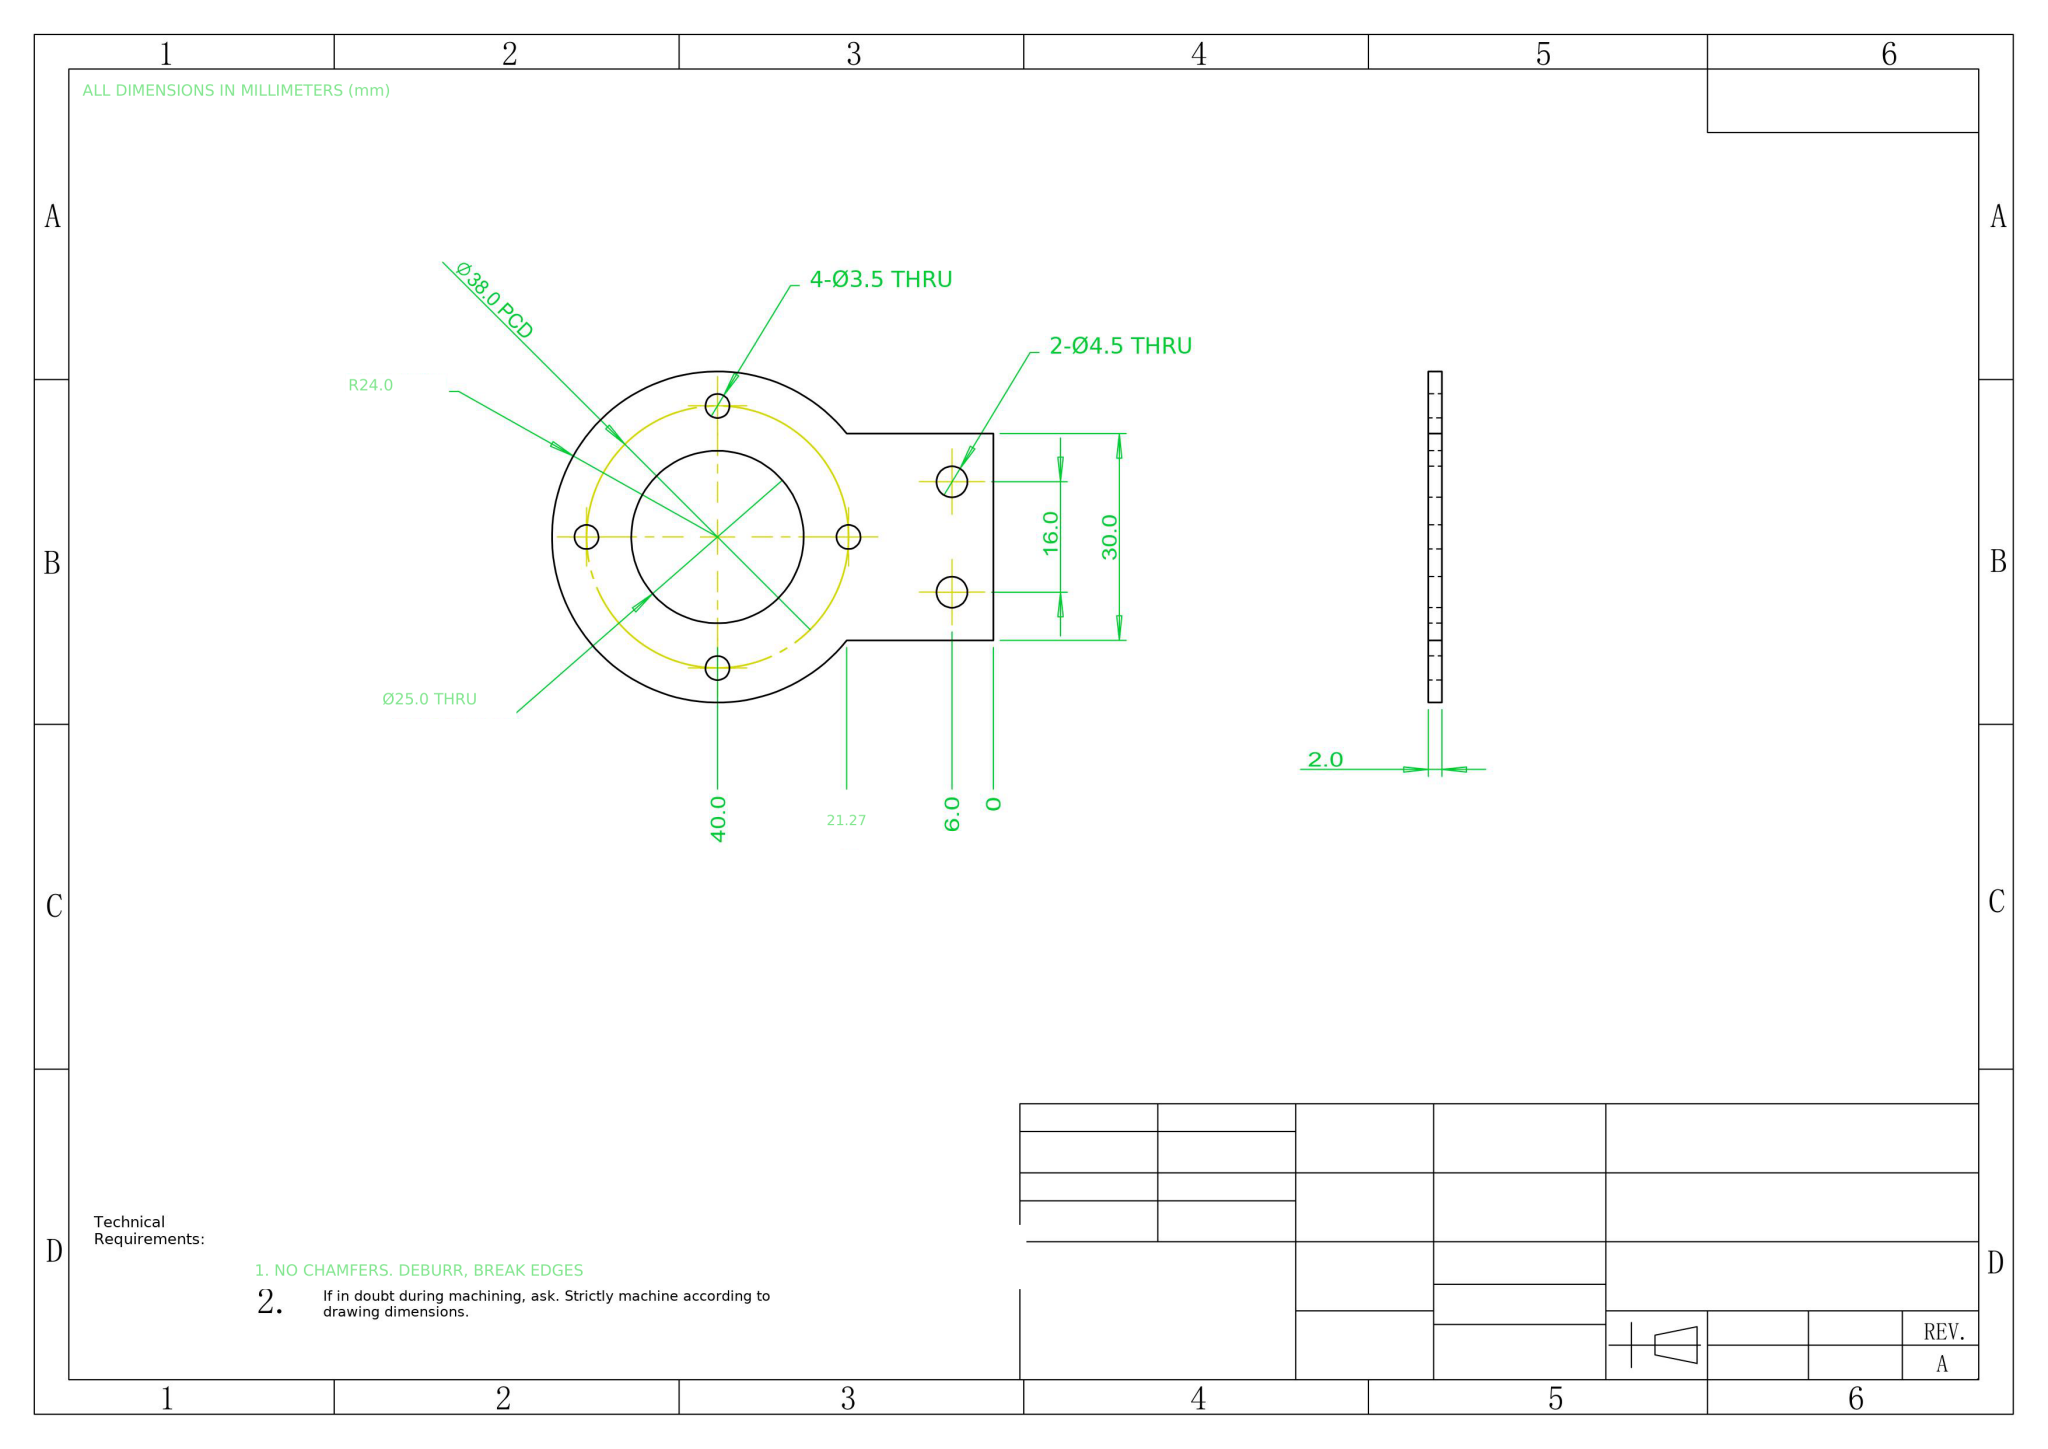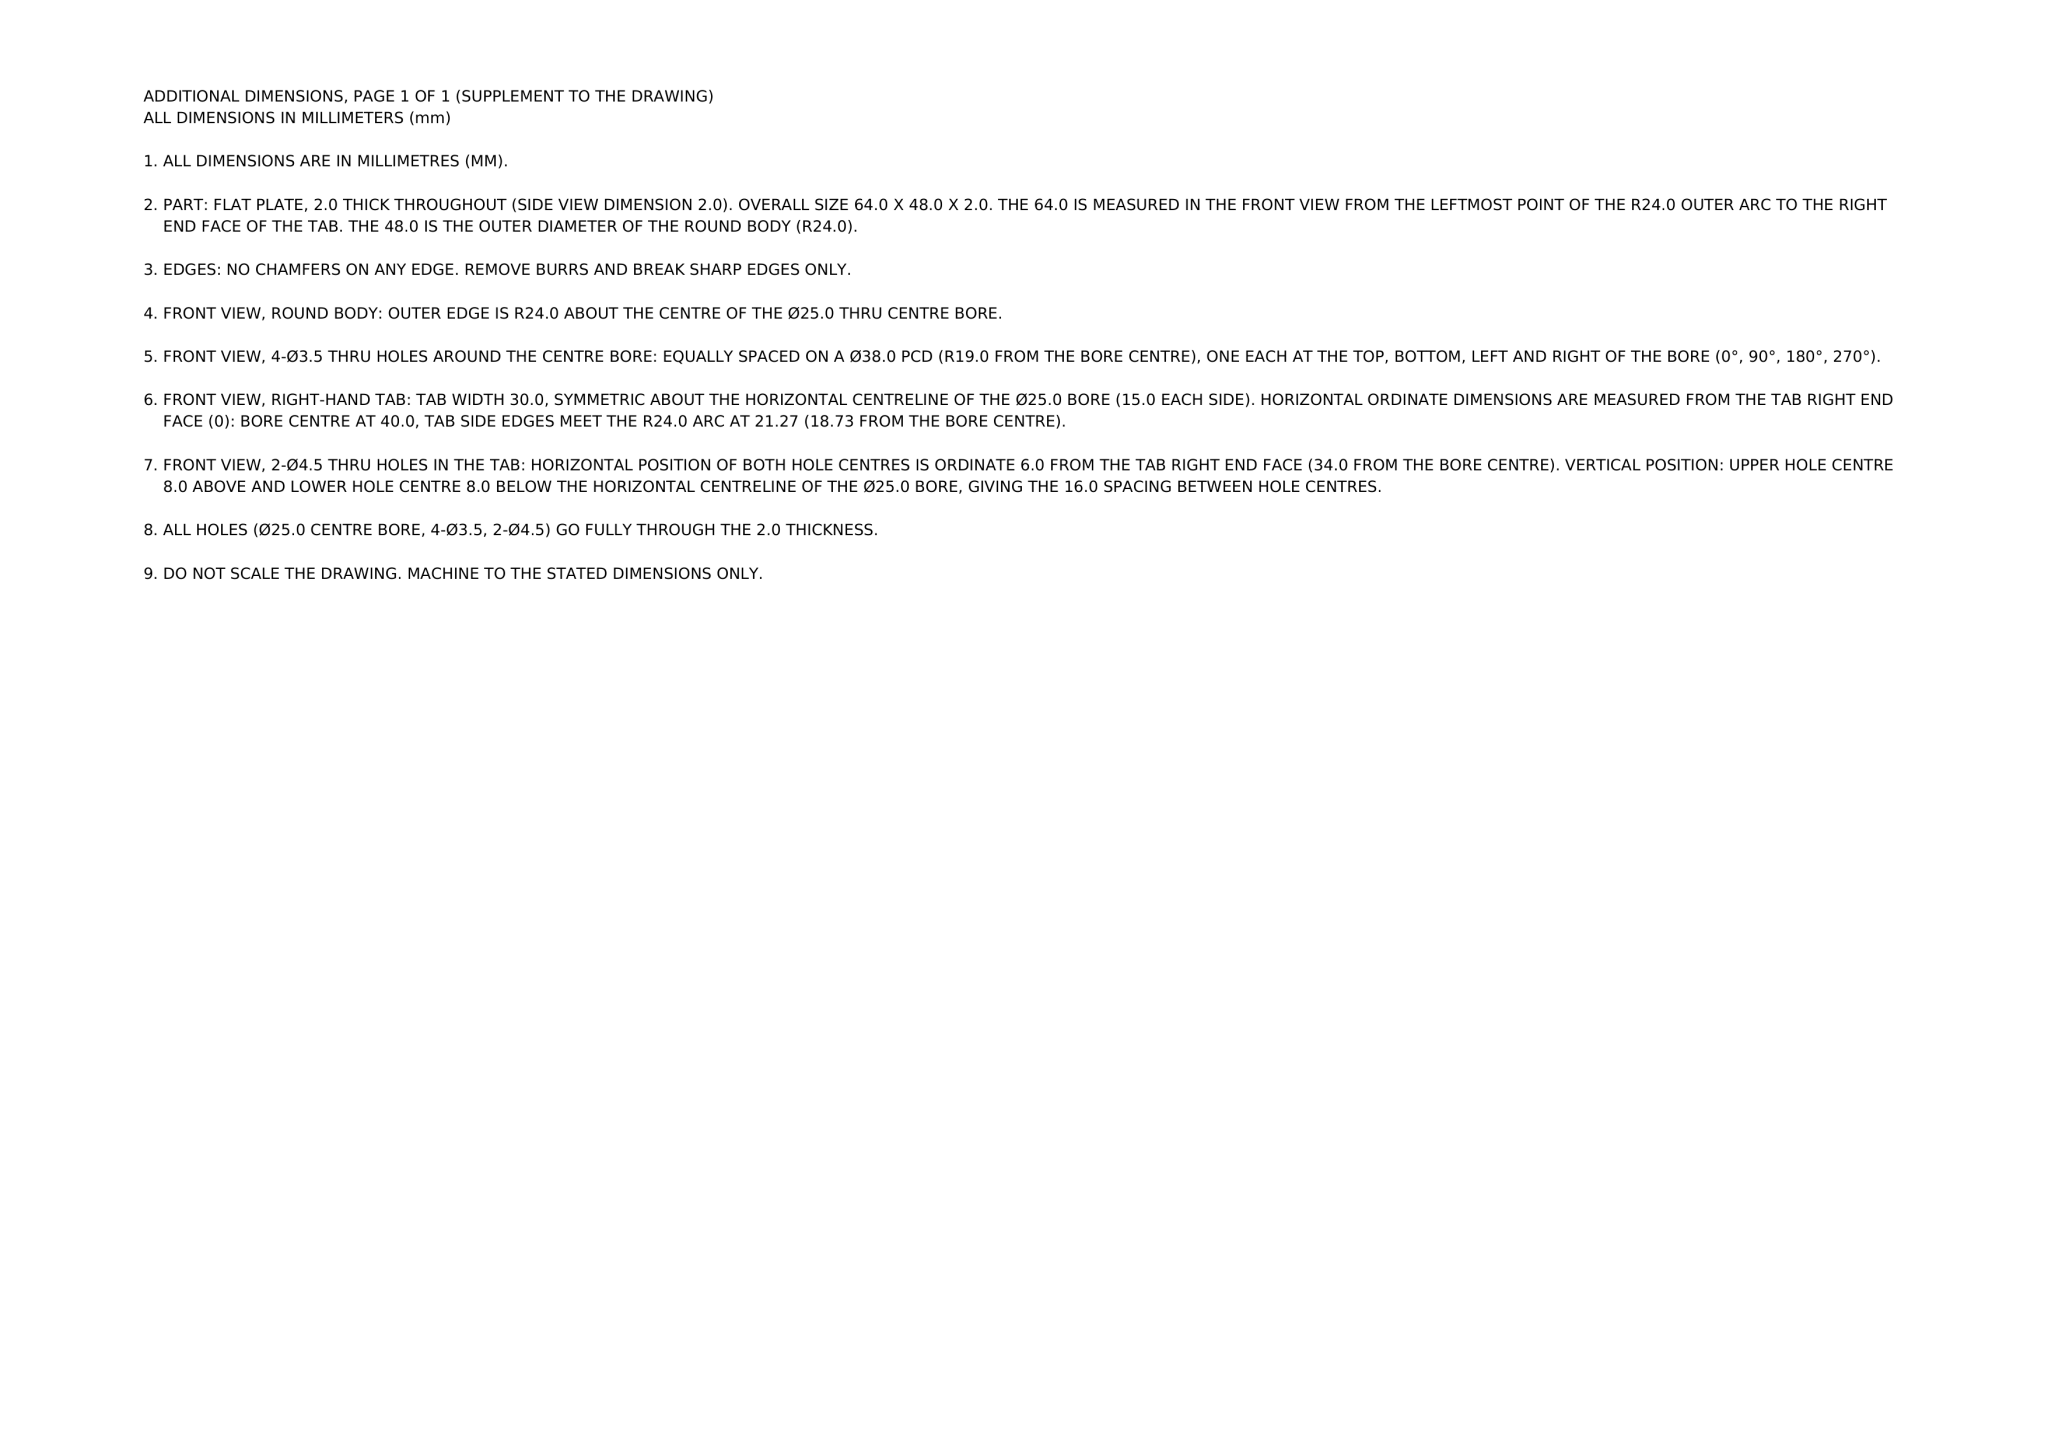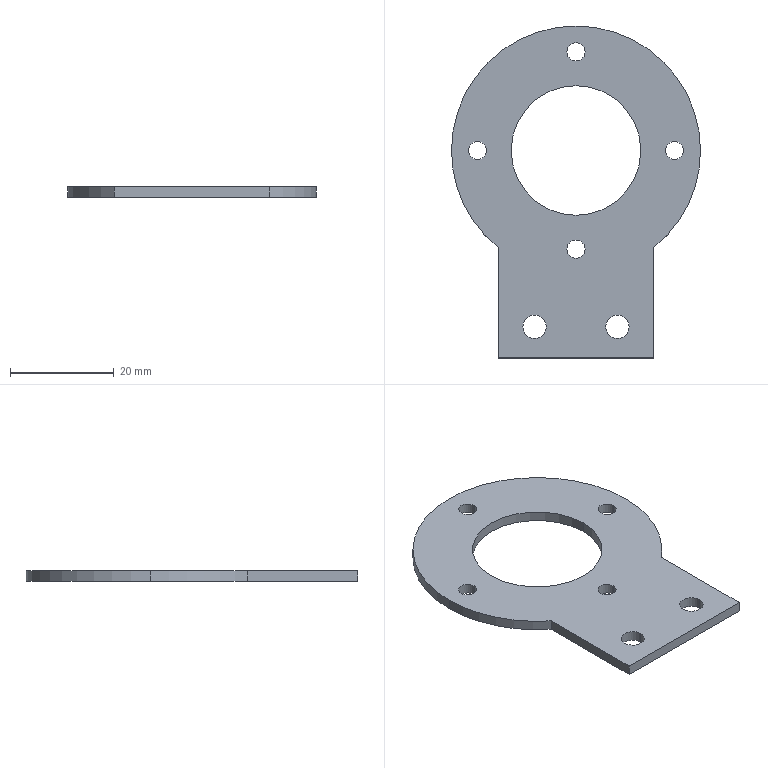Part | NX | mm | 1 solid | 22 faces | box 48 x 64 x 2 mm | volume 3557 mm3 | cylinder 17 | plane 5 | commonest cylinder face diameters 3.5 x8 4.5 x4 48 x3 25 x2
STEP:
#1=COLOUR_RGB('',0.5843,1.,0.);
#2=FILL_AREA_STYLE_COLOUR('',#1);
#3=FILL_AREA_STYLE('',(#2));
#4=SURFACE_STYLE_FILL_AREA(#3);
#5=SURFACE_SIDE_STYLE('',(#4));
#6=SURFACE_STYLE_USAGE(.BOTH.,#5);
#7=PRESENTATION_STYLE_ASSIGNMENT((#6));
#8=CARTESIAN_POINT('',(-10.25,-34.,0.));
#9=VERTEX_POINT('',#8);
#10=CARTESIAN_POINT('',(-5.75,-34.,0.));
#11=VERTEX_POINT('',#10);
#12=CARTESIAN_POINT('',(-8.,-34.,0.));
#13=DIRECTION('',(0.,0.,1.));
#14=DIRECTION('',(1.,0.,0.));
#15=AXIS2_PLACEMENT_3D('',#12,#13,#14);
#16=CIRCLE('',#15,2.25);
#17=EDGE_CURVE('',#9,#11,#16,.T.);
#18=ORIENTED_EDGE('',*,*,#17,.F.);
#19=CARTESIAN_POINT('',(-10.25,-34.,2.));
#20=VERTEX_POINT('',#19);
#21=CARTESIAN_POINT('',(-10.25,-34.,-8.));
#22=DIRECTION('',(0.,0.,1.));
#23=VECTOR('',#22,1000.);
#24=LINE('',#21,#23);
#25=EDGE_CURVE('',#9,#20,#24,.T.);
#26=ORIENTED_EDGE('',*,*,#25,.T.);
#27=CARTESIAN_POINT('',(-5.75,-34.,2.));
#28=VERTEX_POINT('',#27);
#29=CARTESIAN_POINT('',(-8.,-34.,2.));
#30=DIRECTION('',(0.,0.,1.));
#31=DIRECTION('',(-1.,0.,0.));
#32=AXIS2_PLACEMENT_3D('',#29,#30,#31);
#33=CIRCLE('',#32,2.25);
#34=EDGE_CURVE('',#20,#28,#33,.T.);
#35=ORIENTED_EDGE('',*,*,#34,.T.);
#36=CARTESIAN_POINT('',(-5.75,-34.,-8.));
#37=DIRECTION('',(0.,0.,1.));
#38=VECTOR('',#37,1000.);
#39=LINE('',#36,#38);
#40=EDGE_CURVE('',#11,#28,#39,.T.);
#41=ORIENTED_EDGE('',*,*,#40,.F.);
#42=EDGE_LOOP('',(#18,#26,#35,#41));
#43=FACE_OUTER_BOUND('',#42,.T.);
#44=CARTESIAN_POINT('',(-8.,-34.,-8.));
#45=DIRECTION('',(0.,0.,1.));
#46=DIRECTION('',(1.,0.,0.));
#47=AXIS2_PLACEMENT_3D('',#44,#45,#46);
#48=CYLINDRICAL_SURFACE('',#47,2.25);
#49=ADVANCED_FACE('',(#43),#48,.F.);
#50=CARTESIAN_POINT('',(5.75,-34.,0.));
#51=VERTEX_POINT('',#50);
#52=CARTESIAN_POINT('',(10.25,-34.,0.));
#53=VERTEX_POINT('',#52);
#54=CARTESIAN_POINT('',(8.,-34.,0.));
#55=DIRECTION('',(0.,0.,1.));
#56=DIRECTION('',(1.,0.,0.));
#57=AXIS2_PLACEMENT_3D('',#54,#55,#56);
#58=CIRCLE('',#57,2.25);
#59=EDGE_CURVE('',#51,#53,#58,.T.);
#60=ORIENTED_EDGE('',*,*,#59,.F.);
#61=CARTESIAN_POINT('',(5.75,-34.,2.));
#62=VERTEX_POINT('',#61);
#63=CARTESIAN_POINT('',(5.75,-34.,-8.));
#64=DIRECTION('',(0.,0.,1.));
#65=VECTOR('',#64,1000.);
#66=LINE('',#63,#65);
#67=EDGE_CURVE('',#51,#62,#66,.T.);
#68=ORIENTED_EDGE('',*,*,#67,.T.);
#69=CARTESIAN_POINT('',(10.25,-34.,2.));
#70=VERTEX_POINT('',#69);
#71=CARTESIAN_POINT('',(8.,-34.,2.));
#72=DIRECTION('',(0.,0.,1.));
#73=DIRECTION('',(1.,0.,0.));
#74=AXIS2_PLACEMENT_3D('',#71,#72,#73);
#75=CIRCLE('',#74,2.25);
#76=EDGE_CURVE('',#62,#70,#75,.T.);
#77=ORIENTED_EDGE('',*,*,#76,.T.);
#78=CARTESIAN_POINT('',(10.25,-34.,-8.));
#79=DIRECTION('',(0.,0.,1.));
#80=VECTOR('',#79,1000.);
#81=LINE('',#78,#80);
#82=EDGE_CURVE('',#53,#70,#81,.T.);
#83=ORIENTED_EDGE('',*,*,#82,.F.);
#84=EDGE_LOOP('',(#60,#68,#77,#83));
#85=FACE_OUTER_BOUND('',#84,.T.);
#86=CARTESIAN_POINT('',(8.,-34.,-8.));
#87=DIRECTION('',(0.,0.,1.));
#88=DIRECTION('',(1.,0.,0.));
#89=AXIS2_PLACEMENT_3D('',#86,#87,#88);
#90=CYLINDRICAL_SURFACE('',#89,2.25);
#91=ADVANCED_FACE('',(#85),#90,.F.);
#92=CARTESIAN_POINT('',(-20.75,0.,0.));
#93=VERTEX_POINT('',#92);
#94=CARTESIAN_POINT('',(-17.25,0.,0.));
#95=VERTEX_POINT('',#94);
#96=CARTESIAN_POINT('',(-19.,0.,0.));
#97=DIRECTION('',(0.,0.,1.));
#98=DIRECTION('',(1.,0.,0.));
#99=AXIS2_PLACEMENT_3D('',#96,#97,#98);
#100=CIRCLE('',#99,1.75);
#101=EDGE_CURVE('',#93,#95,#100,.T.);
#102=ORIENTED_EDGE('',*,*,#101,.F.);
#103=CARTESIAN_POINT('',(-20.75,0.,2.));
#104=VERTEX_POINT('',#103);
#105=CARTESIAN_POINT('',(-20.75,0.,0.));
#106=DIRECTION('',(0.,0.,1.));
#107=VECTOR('',#106,1000.);
#108=LINE('',#105,#107);
#109=EDGE_CURVE('',#93,#104,#108,.T.);
#110=ORIENTED_EDGE('',*,*,#109,.T.);
#111=CARTESIAN_POINT('',(-17.25,0.,2.));
#112=VERTEX_POINT('',#111);
#113=CARTESIAN_POINT('',(-19.,0.,2.));
#114=DIRECTION('',(0.,0.,1.));
#115=DIRECTION('',(1.,0.,0.));
#116=AXIS2_PLACEMENT_3D('',#113,#114,#115);
#117=CIRCLE('',#116,1.75);
#118=EDGE_CURVE('',#104,#112,#117,.T.);
#119=ORIENTED_EDGE('',*,*,#118,.T.);
#120=CARTESIAN_POINT('',(-17.25,0.,0.));
#121=DIRECTION('',(0.,0.,1.));
#122=VECTOR('',#121,1000.);
#123=LINE('',#120,#122);
#124=EDGE_CURVE('',#95,#112,#123,.T.);
#125=ORIENTED_EDGE('',*,*,#124,.F.);
#126=EDGE_LOOP('',(#102,#110,#119,#125));
#127=FACE_OUTER_BOUND('',#126,.T.);
#128=CARTESIAN_POINT('',(-19.,0.,0.));
#129=DIRECTION('',(0.,0.,1.));
#130=DIRECTION('',(1.,0.,0.));
#131=AXIS2_PLACEMENT_3D('',#128,#129,#130);
#132=CYLINDRICAL_SURFACE('',#131,1.75);
#133=ADVANCED_FACE('',(#127),#132,.F.);
#134=CARTESIAN_POINT('',(-1.75,-19.,0.));
#135=VERTEX_POINT('',#134);
#136=CARTESIAN_POINT('',(1.75,-19.,0.));
#137=VERTEX_POINT('',#136);
#138=CARTESIAN_POINT('',(0.,-19.,0.));
#139=DIRECTION('',(0.,0.,1.));
#140=DIRECTION('',(1.,0.,0.));
#141=AXIS2_PLACEMENT_3D('',#138,#139,#140);
#142=CIRCLE('',#141,1.75);
#143=EDGE_CURVE('',#135,#137,#142,.T.);
#144=ORIENTED_EDGE('',*,*,#143,.F.);
#145=CARTESIAN_POINT('',(-1.75,-19.,2.));
#146=VERTEX_POINT('',#145);
#147=CARTESIAN_POINT('',(-1.75,-19.,0.));
#148=DIRECTION('',(0.,0.,1.));
#149=VECTOR('',#148,1000.);
#150=LINE('',#147,#149);
#151=EDGE_CURVE('',#135,#146,#150,.T.);
#152=ORIENTED_EDGE('',*,*,#151,.T.);
#153=CARTESIAN_POINT('',(1.75,-19.,2.));
#154=VERTEX_POINT('',#153);
#155=CARTESIAN_POINT('',(0.,-19.,2.));
#156=DIRECTION('',(0.,0.,1.));
#157=DIRECTION('',(1.,0.,0.));
#158=AXIS2_PLACEMENT_3D('',#155,#156,#157);
#159=CIRCLE('',#158,1.75);
#160=EDGE_CURVE('',#146,#154,#159,.T.);
#161=ORIENTED_EDGE('',*,*,#160,.T.);
#162=CARTESIAN_POINT('',(1.75,-19.,0.));
#163=DIRECTION('',(0.,0.,1.));
#164=VECTOR('',#163,1000.);
#165=LINE('',#162,#164);
#166=EDGE_CURVE('',#137,#154,#165,.T.);
#167=ORIENTED_EDGE('',*,*,#166,.F.);
#168=EDGE_LOOP('',(#144,#152,#161,#167));
#169=FACE_OUTER_BOUND('',#168,.T.);
#170=CARTESIAN_POINT('',(0.,-19.,0.));
#171=DIRECTION('',(0.,0.,1.));
#172=DIRECTION('',(1.,0.,0.));
#173=AXIS2_PLACEMENT_3D('',#170,#171,#172);
#174=CYLINDRICAL_SURFACE('',#173,1.75);
#175=ADVANCED_FACE('',(#169),#174,.F.);
#176=CARTESIAN_POINT('',(17.25,0.,0.));
#177=VERTEX_POINT('',#176);
#178=CARTESIAN_POINT('',(20.75,0.,0.));
#179=VERTEX_POINT('',#178);
#180=CARTESIAN_POINT('',(19.,0.,0.));
#181=DIRECTION('',(0.,0.,1.));
#182=DIRECTION('',(1.,0.,0.));
#183=AXIS2_PLACEMENT_3D('',#180,#181,#182);
#184=CIRCLE('',#183,1.75);
#185=EDGE_CURVE('',#177,#179,#184,.T.);
#186=ORIENTED_EDGE('',*,*,#185,.F.);
#187=CARTESIAN_POINT('',(17.25,0.,2.));
#188=VERTEX_POINT('',#187);
#189=CARTESIAN_POINT('',(17.25,0.,0.));
#190=DIRECTION('',(0.,0.,1.));
#191=VECTOR('',#190,1000.);
#192=LINE('',#189,#191);
#193=EDGE_CURVE('',#177,#188,#192,.T.);
#194=ORIENTED_EDGE('',*,*,#193,.T.);
#195=CARTESIAN_POINT('',(20.75,0.,2.));
#196=VERTEX_POINT('',#195);
#197=CARTESIAN_POINT('',(19.,0.,2.));
#198=DIRECTION('',(0.,0.,1.));
#199=DIRECTION('',(1.,0.,0.));
#200=AXIS2_PLACEMENT_3D('',#197,#198,#199);
#201=CIRCLE('',#200,1.75);
#202=EDGE_CURVE('',#188,#196,#201,.T.);
#203=ORIENTED_EDGE('',*,*,#202,.T.);
#204=CARTESIAN_POINT('',(20.75,0.,0.));
#205=DIRECTION('',(0.,0.,1.));
#206=VECTOR('',#205,1000.);
#207=LINE('',#204,#206);
#208=EDGE_CURVE('',#179,#196,#207,.T.);
#209=ORIENTED_EDGE('',*,*,#208,.F.);
#210=EDGE_LOOP('',(#186,#194,#203,#209));
#211=FACE_OUTER_BOUND('',#210,.T.);
#212=CARTESIAN_POINT('',(19.,0.,0.));
#213=DIRECTION('',(0.,0.,1.));
#214=DIRECTION('',(1.,0.,0.));
#215=AXIS2_PLACEMENT_3D('',#212,#213,#214);
#216=CYLINDRICAL_SURFACE('',#215,1.75);
#217=ADVANCED_FACE('',(#211),#216,.F.);
#218=CARTESIAN_POINT('',(-1.75,19.,0.));
#219=VERTEX_POINT('',#218);
#220=CARTESIAN_POINT('',(1.75,19.,0.));
#221=VERTEX_POINT('',#220);
#222=CARTESIAN_POINT('',(0.,19.,0.));
#223=DIRECTION('',(0.,0.,1.));
#224=DIRECTION('',(1.,0.,0.));
#225=AXIS2_PLACEMENT_3D('',#222,#223,#224);
#226=CIRCLE('',#225,1.75);
#227=EDGE_CURVE('',#219,#221,#226,.T.);
#228=ORIENTED_EDGE('',*,*,#227,.F.);
#229=CARTESIAN_POINT('',(-1.75,19.,2.));
#230=VERTEX_POINT('',#229);
#231=CARTESIAN_POINT('',(-1.75,19.,0.));
#232=DIRECTION('',(0.,0.,1.));
#233=VECTOR('',#232,1000.);
#234=LINE('',#231,#233);
#235=EDGE_CURVE('',#219,#230,#234,.T.);
#236=ORIENTED_EDGE('',*,*,#235,.T.);
#237=CARTESIAN_POINT('',(1.75,19.,2.));
#238=VERTEX_POINT('',#237);
#239=CARTESIAN_POINT('',(0.,19.,2.));
#240=DIRECTION('',(0.,0.,1.));
#241=DIRECTION('',(1.,0.,0.));
#242=AXIS2_PLACEMENT_3D('',#239,#240,#241);
#243=CIRCLE('',#242,1.75);
#244=EDGE_CURVE('',#230,#238,#243,.T.);
#245=ORIENTED_EDGE('',*,*,#244,.T.);
#246=CARTESIAN_POINT('',(1.75,19.,0.));
#247=DIRECTION('',(0.,0.,1.));
#248=VECTOR('',#247,1000.);
#249=LINE('',#246,#248);
#250=EDGE_CURVE('',#221,#238,#249,.T.);
#251=ORIENTED_EDGE('',*,*,#250,.F.);
#252=EDGE_LOOP('',(#228,#236,#245,#251));
#253=FACE_OUTER_BOUND('',#252,.T.);
#254=CARTESIAN_POINT('',(0.,19.,0.));
#255=DIRECTION('',(0.,0.,1.));
#256=DIRECTION('',(1.,0.,0.));
#257=AXIS2_PLACEMENT_3D('',#254,#255,#256);
#258=CYLINDRICAL_SURFACE('',#257,1.75);
#259=ADVANCED_FACE('',(#253),#258,.F.);
#260=CARTESIAN_POINT('',(-12.5,0.,2.));
#261=VERTEX_POINT('',#260);
#262=CARTESIAN_POINT('',(12.5,0.,2.));
#263=VERTEX_POINT('',#262);
#264=CARTESIAN_POINT('',(0.,0.,2.));
#265=DIRECTION('',(0.,0.,1.));
#266=DIRECTION('',(1.,0.,0.));
#267=AXIS2_PLACEMENT_3D('',#264,#265,#266);
#268=CIRCLE('',#267,12.5);
#269=EDGE_CURVE('',#261,#263,#268,.T.);
#270=ORIENTED_EDGE('',*,*,#269,.T.);
#271=CARTESIAN_POINT('',(12.5,0.,0.));
#272=VERTEX_POINT('',#271);
#273=CARTESIAN_POINT('',(12.5,0.,2.));
#274=DIRECTION('',(0.,0.,-1.));
#275=VECTOR('',#274,1000.);
#276=LINE('',#273,#275);
#277=EDGE_CURVE('',#263,#272,#276,.T.);
#278=ORIENTED_EDGE('',*,*,#277,.T.);
#279=CARTESIAN_POINT('',(-12.5,0.,0.));
#280=VERTEX_POINT('',#279);
#281=CARTESIAN_POINT('',(0.,0.,0.));
#282=DIRECTION('',(0.,0.,1.));
#283=DIRECTION('',(1.,0.,0.));
#284=AXIS2_PLACEMENT_3D('',#281,#282,#283);
#285=CIRCLE('',#284,12.5);
#286=EDGE_CURVE('',#280,#272,#285,.T.);
#287=ORIENTED_EDGE('',*,*,#286,.F.);
#288=CARTESIAN_POINT('',(-12.5,0.,2.));
#289=DIRECTION('',(0.,0.,-1.));
#290=VECTOR('',#289,1000.);
#291=LINE('',#288,#290);
#292=EDGE_CURVE('',#261,#280,#291,.T.);
#293=ORIENTED_EDGE('',*,*,#292,.F.);
#294=EDGE_LOOP('',(#270,#278,#287,#293));
#295=FACE_OUTER_BOUND('',#294,.T.);
#296=CARTESIAN_POINT('',(0.,0.,2.));
#297=DIRECTION('',(0.,0.,-1.));
#298=DIRECTION('',(-1.,0.,0.));
#299=AXIS2_PLACEMENT_3D('',#296,#297,#298);
#300=CYLINDRICAL_SURFACE('',#299,12.5);
#301=ADVANCED_FACE('',(#295),#300,.F.);
#302=CARTESIAN_POINT('',(24.,0.,2.));
#303=VERTEX_POINT('',#302);
#304=CARTESIAN_POINT('',(-24.,0.,2.));
#305=VERTEX_POINT('',#304);
#306=CARTESIAN_POINT('',(0.,0.,2.));
#307=DIRECTION('',(0.,0.,1.));
#308=DIRECTION('',(1.,0.,0.));
#309=AXIS2_PLACEMENT_3D('',#306,#307,#308);
#310=CIRCLE('',#309,24.);
#311=EDGE_CURVE('',#303,#305,#310,.T.);
#312=ORIENTED_EDGE('',*,*,#311,.F.);
#313=CARTESIAN_POINT('',(24.,0.,0.));
#314=VERTEX_POINT('',#313);
#315=CARTESIAN_POINT('',(24.,0.,2.));
#316=DIRECTION('',(0.,0.,-1.));
#317=VECTOR('',#316,1000.);
#318=LINE('',#315,#317);
#319=EDGE_CURVE('',#303,#314,#318,.T.);
#320=ORIENTED_EDGE('',*,*,#319,.T.);
#321=CARTESIAN_POINT('',(-24.,0.,0.));
#322=VERTEX_POINT('',#321);
#323=CARTESIAN_POINT('',(0.,0.,0.));
#324=DIRECTION('',(0.,0.,1.));
#325=DIRECTION('',(1.,0.,0.));
#326=AXIS2_PLACEMENT_3D('',#323,#324,#325);
#327=CIRCLE('',#326,24.);
#328=EDGE_CURVE('',#314,#322,#327,.T.);
#329=ORIENTED_EDGE('',*,*,#328,.T.);
#330=CARTESIAN_POINT('',(-24.,0.,2.));
#331=DIRECTION('',(0.,0.,-1.));
#332=VECTOR('',#331,1000.);
#333=LINE('',#330,#332);
#334=EDGE_CURVE('',#305,#322,#333,.T.);
#335=ORIENTED_EDGE('',*,*,#334,.F.);
#336=EDGE_LOOP('',(#312,#320,#329,#335));
#337=FACE_OUTER_BOUND('',#336,.T.);
#338=CARTESIAN_POINT('',(0.,0.,2.));
#339=DIRECTION('',(0.,0.,-1.));
#340=DIRECTION('',(-1.,0.,0.));
#341=AXIS2_PLACEMENT_3D('',#338,#339,#340);
#342=CYLINDRICAL_SURFACE('',#341,24.);
#343=ADVANCED_FACE('',(#337),#342,.T.);
#344=CARTESIAN_POINT('',(-15.,-18.735,2.));
#345=VERTEX_POINT('',#344);
#346=CARTESIAN_POINT('',(0.,0.,2.));
#347=DIRECTION('',(0.,0.,1.));
#348=DIRECTION('',(1.,0.,0.));
#349=AXIS2_PLACEMENT_3D('',#346,#347,#348);
#350=CIRCLE('',#349,24.);
#351=EDGE_CURVE('',#305,#345,#350,.T.);
#352=ORIENTED_EDGE('',*,*,#351,.F.);
#353=ORIENTED_EDGE('',*,*,#334,.T.);
#354=CARTESIAN_POINT('',(-15.,-18.735,0.));
#355=VERTEX_POINT('',#354);
#356=CARTESIAN_POINT('',(0.,0.,0.));
#357=DIRECTION('',(0.,0.,1.));
#358=DIRECTION('',(1.,0.,0.));
#359=AXIS2_PLACEMENT_3D('',#356,#357,#358);
#360=CIRCLE('',#359,24.);
#361=EDGE_CURVE('',#322,#355,#360,.T.);
#362=ORIENTED_EDGE('',*,*,#361,.T.);
#363=CARTESIAN_POINT('',(-15.,-18.735,2.));
#364=DIRECTION('',(0.,0.,1.));
#365=VECTOR('',#364,1000.);
#366=LINE('',#363,#365);
#367=EDGE_CURVE('',#355,#345,#366,.T.);
#368=ORIENTED_EDGE('',*,*,#367,.T.);
#369=EDGE_LOOP('',(#352,#353,#362,#368));
#370=FACE_OUTER_BOUND('',#369,.T.);
#371=CARTESIAN_POINT('',(0.,0.,2.));
#372=DIRECTION('',(0.,0.,-1.));
#373=DIRECTION('',(-1.,0.,0.));
#374=AXIS2_PLACEMENT_3D('',#371,#372,#373);
#375=CYLINDRICAL_SURFACE('',#374,24.);
#376=ADVANCED_FACE('',(#370),#375,.T.);
#377=CARTESIAN_POINT('',(-8.,-34.,2.));
#378=DIRECTION('',(0.,0.,1.));
#379=DIRECTION('',(-1.,0.,0.));
#380=AXIS2_PLACEMENT_3D('',#377,#378,#379);
#381=CIRCLE('',#380,2.25);
#382=EDGE_CURVE('',#28,#20,#381,.T.);
#383=ORIENTED_EDGE('',*,*,#382,.F.);
#384=ORIENTED_EDGE('',*,*,#34,.F.);
#385=EDGE_LOOP('',(#383,#384));
#386=FACE_BOUND('',#385,.T.);
#387=CARTESIAN_POINT('',(8.,-34.,2.));
#388=DIRECTION('',(0.,0.,1.));
#389=DIRECTION('',(1.,0.,0.));
#390=AXIS2_PLACEMENT_3D('',#387,#388,#389);
#391=CIRCLE('',#390,2.25);
#392=EDGE_CURVE('',#70,#62,#391,.T.);
#393=ORIENTED_EDGE('',*,*,#392,.F.);
#394=ORIENTED_EDGE('',*,*,#76,.F.);
#395=EDGE_LOOP('',(#393,#394));
#396=FACE_BOUND('',#395,.T.);
#397=CARTESIAN_POINT('',(-19.,0.,2.));
#398=DIRECTION('',(0.,0.,1.));
#399=DIRECTION('',(1.,0.,0.));
#400=AXIS2_PLACEMENT_3D('',#397,#398,#399);
#401=CIRCLE('',#400,1.75);
#402=EDGE_CURVE('',#112,#104,#401,.T.);
#403=ORIENTED_EDGE('',*,*,#402,.F.);
#404=ORIENTED_EDGE('',*,*,#118,.F.);
#405=EDGE_LOOP('',(#403,#404));
#406=FACE_BOUND('',#405,.T.);
#407=CARTESIAN_POINT('',(0.,-19.,2.));
#408=DIRECTION('',(0.,0.,1.));
#409=DIRECTION('',(1.,0.,0.));
#410=AXIS2_PLACEMENT_3D('',#407,#408,#409);
#411=CIRCLE('',#410,1.75);
#412=EDGE_CURVE('',#154,#146,#411,.T.);
#413=ORIENTED_EDGE('',*,*,#412,.F.);
#414=ORIENTED_EDGE('',*,*,#160,.F.);
#415=EDGE_LOOP('',(#413,#414));
#416=FACE_BOUND('',#415,.T.);
#417=CARTESIAN_POINT('',(19.,0.,2.));
#418=DIRECTION('',(0.,0.,1.));
#419=DIRECTION('',(1.,0.,0.));
#420=AXIS2_PLACEMENT_3D('',#417,#418,#419);
#421=CIRCLE('',#420,1.75);
#422=EDGE_CURVE('',#196,#188,#421,.T.);
#423=ORIENTED_EDGE('',*,*,#422,.F.);
#424=ORIENTED_EDGE('',*,*,#202,.F.);
#425=EDGE_LOOP('',(#423,#424));
#426=FACE_BOUND('',#425,.T.);
#427=CARTESIAN_POINT('',(0.,19.,2.));
#428=DIRECTION('',(0.,0.,1.));
#429=DIRECTION('',(1.,0.,0.));
#430=AXIS2_PLACEMENT_3D('',#427,#428,#429);
#431=CIRCLE('',#430,1.75);
#432=EDGE_CURVE('',#238,#230,#431,.T.);
#433=ORIENTED_EDGE('',*,*,#432,.F.);
#434=ORIENTED_EDGE('',*,*,#244,.F.);
#435=EDGE_LOOP('',(#433,#434));
#436=FACE_BOUND('',#435,.T.);
#437=CARTESIAN_POINT('',(15.,-18.735,2.));
#438=VERTEX_POINT('',#437);
#439=CARTESIAN_POINT('',(0.,0.,2.));
#440=DIRECTION('',(0.,0.,1.));
#441=DIRECTION('',(1.,0.,0.));
#442=AXIS2_PLACEMENT_3D('',#439,#440,#441);
#443=CIRCLE('',#442,24.);
#444=EDGE_CURVE('',#438,#303,#443,.T.);
#445=ORIENTED_EDGE('',*,*,#444,.T.);
#446=ORIENTED_EDGE('',*,*,#311,.T.);
#447=ORIENTED_EDGE('',*,*,#351,.T.);
#448=CARTESIAN_POINT('',(-15.,-40.,2.));
#449=VERTEX_POINT('',#448);
#450=CARTESIAN_POINT('',(-15.,-15.209,2.));
#451=DIRECTION('',(0.,-1.,0.));
#452=VECTOR('',#451,1000.);
#453=LINE('',#450,#452);
#454=EDGE_CURVE('',#345,#449,#453,.T.);
#455=ORIENTED_EDGE('',*,*,#454,.T.);
#456=CARTESIAN_POINT('',(15.,-40.,2.));
#457=VERTEX_POINT('',#456);
#458=CARTESIAN_POINT('',(-15.,-40.,2.));
#459=DIRECTION('',(1.,0.,0.));
#460=VECTOR('',#459,1000.);
#461=LINE('',#458,#460);
#462=EDGE_CURVE('',#449,#457,#461,.T.);
#463=ORIENTED_EDGE('',*,*,#462,.T.);
#464=CARTESIAN_POINT('',(15.,-15.209,2.));
#465=DIRECTION('',(-0.,1.,0.));
#466=VECTOR('',#465,1000.);
#467=LINE('',#464,#466);
#468=EDGE_CURVE('',#457,#438,#467,.T.);
#469=ORIENTED_EDGE('',*,*,#468,.T.);
#470=EDGE_LOOP('',(#445,#446,#447,#455,#463,#469));
#471=FACE_OUTER_BOUND('',#470,.T.);
#472=ORIENTED_EDGE('',*,*,#269,.F.);
#473=CARTESIAN_POINT('',(0.,0.,2.));
#474=DIRECTION('',(0.,0.,1.));
#475=DIRECTION('',(1.,0.,0.));
#476=AXIS2_PLACEMENT_3D('',#473,#474,#475);
#477=CIRCLE('',#476,12.5);
#478=EDGE_CURVE('',#263,#261,#477,.T.);
#479=ORIENTED_EDGE('',*,*,#478,.F.);
#480=EDGE_LOOP('',(#472,#479));
#481=FACE_BOUND('',#480,.T.);
#482=CARTESIAN_POINT('',(0.,0.,2.));
#483=DIRECTION('',(0.,0.,1.));
#484=DIRECTION('',(1.,0.,0.));
#485=AXIS2_PLACEMENT_3D('',#482,#483,#484);
#486=PLANE('',#485);
#487=ADVANCED_FACE('',(#386,#396,#406,#416,#426,#436,#471,#481),#486,.T.);
#488=CARTESIAN_POINT('',(-8.,-34.,0.));
#489=DIRECTION('',(0.,0.,1.));
#490=DIRECTION('',(1.,0.,0.));
#491=AXIS2_PLACEMENT_3D('',#488,#489,#490);
#492=CIRCLE('',#491,2.25);
#493=EDGE_CURVE('',#11,#9,#492,.T.);
#494=ORIENTED_EDGE('',*,*,#493,.T.);
#495=ORIENTED_EDGE('',*,*,#17,.T.);
#496=EDGE_LOOP('',(#494,#495));
#497=FACE_BOUND('',#496,.T.);
#498=CARTESIAN_POINT('',(8.,-34.,0.));
#499=DIRECTION('',(0.,0.,1.));
#500=DIRECTION('',(1.,0.,0.));
#501=AXIS2_PLACEMENT_3D('',#498,#499,#500);
#502=CIRCLE('',#501,2.25);
#503=EDGE_CURVE('',#53,#51,#502,.T.);
#504=ORIENTED_EDGE('',*,*,#503,.T.);
#505=ORIENTED_EDGE('',*,*,#59,.T.);
#506=EDGE_LOOP('',(#504,#505));
#507=FACE_BOUND('',#506,.T.);
#508=CARTESIAN_POINT('',(-19.,0.,0.));
#509=DIRECTION('',(0.,0.,1.));
#510=DIRECTION('',(1.,0.,0.));
#511=AXIS2_PLACEMENT_3D('',#508,#509,#510);
#512=CIRCLE('',#511,1.75);
#513=EDGE_CURVE('',#95,#93,#512,.T.);
#514=ORIENTED_EDGE('',*,*,#513,.T.);
#515=ORIENTED_EDGE('',*,*,#101,.T.);
#516=EDGE_LOOP('',(#514,#515));
#517=FACE_BOUND('',#516,.T.);
#518=CARTESIAN_POINT('',(0.,-19.,0.));
#519=DIRECTION('',(0.,0.,1.));
#520=DIRECTION('',(1.,0.,0.));
#521=AXIS2_PLACEMENT_3D('',#518,#519,#520);
#522=CIRCLE('',#521,1.75);
#523=EDGE_CURVE('',#137,#135,#522,.T.);
#524=ORIENTED_EDGE('',*,*,#523,.T.);
#525=ORIENTED_EDGE('',*,*,#143,.T.);
#526=EDGE_LOOP('',(#524,#525));
#527=FACE_BOUND('',#526,.T.);
#528=CARTESIAN_POINT('',(19.,0.,0.));
#529=DIRECTION('',(0.,0.,1.));
#530=DIRECTION('',(1.,0.,0.));
#531=AXIS2_PLACEMENT_3D('',#528,#529,#530);
#532=CIRCLE('',#531,1.75);
#533=EDGE_CURVE('',#179,#177,#532,.T.);
#534=ORIENTED_EDGE('',*,*,#533,.T.);
#535=ORIENTED_EDGE('',*,*,#185,.T.);
#536=EDGE_LOOP('',(#534,#535));
#537=FACE_BOUND('',#536,.T.);
#538=CARTESIAN_POINT('',(0.,19.,0.));
#539=DIRECTION('',(0.,0.,1.));
#540=DIRECTION('',(1.,0.,0.));
#541=AXIS2_PLACEMENT_3D('',#538,#539,#540);
#542=CIRCLE('',#541,1.75);
#543=EDGE_CURVE('',#221,#219,#542,.T.);
#544=ORIENTED_EDGE('',*,*,#543,.T.);
#545=ORIENTED_EDGE('',*,*,#227,.T.);
#546=EDGE_LOOP('',(#544,#545));
#547=FACE_BOUND('',#546,.T.);
#548=CARTESIAN_POINT('',(-15.,-40.,0.));
#549=VERTEX_POINT('',#548);
#550=CARTESIAN_POINT('',(-15.,-15.209,0.));
#551=DIRECTION('',(-0.,1.,0.));
#552=VECTOR('',#551,1000.);
#553=LINE('',#550,#552);
#554=EDGE_CURVE('',#549,#355,#553,.T.);
#555=ORIENTED_EDGE('',*,*,#554,.T.);
#556=ORIENTED_EDGE('',*,*,#361,.F.);
#557=ORIENTED_EDGE('',*,*,#328,.F.);
#558=CARTESIAN_POINT('',(15.,-18.735,0.));
#559=VERTEX_POINT('',#558);
#560=CARTESIAN_POINT('',(0.,0.,0.));
#561=DIRECTION('',(0.,0.,1.));
#562=DIRECTION('',(1.,0.,0.));
#563=AXIS2_PLACEMENT_3D('',#560,#561,#562);
#564=CIRCLE('',#563,24.);
#565=EDGE_CURVE('',#559,#314,#564,.T.);
#566=ORIENTED_EDGE('',*,*,#565,.F.);
#567=CARTESIAN_POINT('',(15.,-40.,0.));
#568=VERTEX_POINT('',#567);
#569=CARTESIAN_POINT('',(15.,-15.209,0.));
#570=DIRECTION('',(0.,-1.,0.));
#571=VECTOR('',#570,1000.);
#572=LINE('',#569,#571);
#573=EDGE_CURVE('',#559,#568,#572,.T.);
#574=ORIENTED_EDGE('',*,*,#573,.T.);
#575=CARTESIAN_POINT('',(-15.,-40.,0.));
#576=DIRECTION('',(-1.,0.,0.));
#577=VECTOR('',#576,1000.);
#578=LINE('',#575,#577);
#579=EDGE_CURVE('',#568,#549,#578,.T.);
#580=ORIENTED_EDGE('',*,*,#579,.T.);
#581=EDGE_LOOP('',(#555,#556,#557,#566,#574,#580));
#582=FACE_OUTER_BOUND('',#581,.T.);
#583=ORIENTED_EDGE('',*,*,#286,.T.);
#584=CARTESIAN_POINT('',(0.,0.,0.));
#585=DIRECTION('',(0.,0.,1.));
#586=DIRECTION('',(1.,0.,0.));
#587=AXIS2_PLACEMENT_3D('',#584,#585,#586);
#588=CIRCLE('',#587,12.5);
#589=EDGE_CURVE('',#272,#280,#588,.T.);
#590=ORIENTED_EDGE('',*,*,#589,.T.);
#591=EDGE_LOOP('',(#583,#590));
#592=FACE_BOUND('',#591,.T.);
#593=CARTESIAN_POINT('',(0.,0.,0.));
#594=DIRECTION('',(0.,0.,1.));
#595=DIRECTION('',(1.,0.,0.));
#596=AXIS2_PLACEMENT_3D('',#593,#594,#595);
#597=PLANE('',#596);
#598=ADVANCED_FACE('',(#497,#507,#517,#527,#537,#547,#582,#592),#597,.F.);
#599=ORIENTED_EDGE('',*,*,#319,.F.);
#600=ORIENTED_EDGE('',*,*,#444,.F.);
#601=CARTESIAN_POINT('',(15.,-18.735,2.));
#602=DIRECTION('',(0.,0.,-1.));
#603=VECTOR('',#602,1000.);
#604=LINE('',#601,#603);
#605=EDGE_CURVE('',#438,#559,#604,.T.);
#606=ORIENTED_EDGE('',*,*,#605,.T.);
#607=ORIENTED_EDGE('',*,*,#565,.T.);
#608=EDGE_LOOP('',(#599,#600,#606,#607));
#609=FACE_OUTER_BOUND('',#608,.T.);
#610=CARTESIAN_POINT('',(0.,0.,2.));
#611=DIRECTION('',(0.,0.,-1.));
#612=DIRECTION('',(-1.,0.,0.));
#613=AXIS2_PLACEMENT_3D('',#610,#611,#612);
#614=CYLINDRICAL_SURFACE('',#613,24.);
#615=ADVANCED_FACE('',(#609),#614,.T.);
#616=ORIENTED_EDGE('',*,*,#277,.F.);
#617=ORIENTED_EDGE('',*,*,#478,.T.);
#618=ORIENTED_EDGE('',*,*,#292,.T.);
#619=ORIENTED_EDGE('',*,*,#589,.F.);
#620=EDGE_LOOP('',(#616,#617,#618,#619));
#621=FACE_OUTER_BOUND('',#620,.T.);
#622=CARTESIAN_POINT('',(0.,0.,2.));
#623=DIRECTION('',(0.,0.,-1.));
#624=DIRECTION('',(-1.,0.,0.));
#625=AXIS2_PLACEMENT_3D('',#622,#623,#624);
#626=CYLINDRICAL_SURFACE('',#625,12.5);
#627=ADVANCED_FACE('',(#621),#626,.F.);
#628=ORIENTED_EDGE('',*,*,#605,.F.);
#629=ORIENTED_EDGE('',*,*,#468,.F.);
#630=CARTESIAN_POINT('',(15.,-40.,-38.918));
#631=DIRECTION('',(0.,0.,1.));
#632=VECTOR('',#631,1000.);
#633=LINE('',#630,#632);
#634=EDGE_CURVE('',#568,#457,#633,.T.);
#635=ORIENTED_EDGE('',*,*,#634,.F.);
#636=ORIENTED_EDGE('',*,*,#573,.F.);
#637=EDGE_LOOP('',(#628,#629,#635,#636));
#638=FACE_OUTER_BOUND('',#637,.T.);
#639=CARTESIAN_POINT('',(15.,-15.209,-38.918));
#640=DIRECTION('',(1.,0.,0.));
#641=DIRECTION('',(-0.,1.,0.));
#642=AXIS2_PLACEMENT_3D('',#639,#640,#641);
#643=PLANE('',#642);
#644=ADVANCED_FACE('',(#638),#643,.T.);
#645=ORIENTED_EDGE('',*,*,#367,.F.);
#646=ORIENTED_EDGE('',*,*,#554,.F.);
#647=CARTESIAN_POINT('',(-15.,-40.,-38.918));
#648=DIRECTION('',(0.,0.,1.));
#649=VECTOR('',#648,1000.);
#650=LINE('',#647,#649);
#651=EDGE_CURVE('',#549,#449,#650,.T.);
#652=ORIENTED_EDGE('',*,*,#651,.T.);
#653=ORIENTED_EDGE('',*,*,#454,.F.);
#654=EDGE_LOOP('',(#645,#646,#652,#653));
#655=FACE_OUTER_BOUND('',#654,.T.);
#656=CARTESIAN_POINT('',(-15.,-15.209,-38.918));
#657=DIRECTION('',(-1.,-0.,0.));
#658=DIRECTION('',(0.,-1.,0.));
#659=AXIS2_PLACEMENT_3D('',#656,#657,#658);
#660=PLANE('',#659);
#661=ADVANCED_FACE('',(#655),#660,.T.);
#662=ORIENTED_EDGE('',*,*,#579,.F.);
#663=ORIENTED_EDGE('',*,*,#634,.T.);
#664=ORIENTED_EDGE('',*,*,#462,.F.);
#665=ORIENTED_EDGE('',*,*,#651,.F.);
#666=EDGE_LOOP('',(#662,#663,#664,#665));
#667=FACE_OUTER_BOUND('',#666,.T.);
#668=CARTESIAN_POINT('',(-15.,-40.,-38.918));
#669=DIRECTION('',(0.,-1.,0.));
#670=DIRECTION('',(0.,0.,-1.));
#671=AXIS2_PLACEMENT_3D('',#668,#669,#670);
#672=PLANE('',#671);
#673=ADVANCED_FACE('',(#667),#672,.T.);
#674=ORIENTED_EDGE('',*,*,#235,.F.);
#675=ORIENTED_EDGE('',*,*,#543,.F.);
#676=ORIENTED_EDGE('',*,*,#250,.T.);
#677=ORIENTED_EDGE('',*,*,#432,.T.);
#678=EDGE_LOOP('',(#674,#675,#676,#677));
#679=FACE_OUTER_BOUND('',#678,.T.);
#680=CARTESIAN_POINT('',(0.,19.,0.));
#681=DIRECTION('',(0.,0.,1.));
#682=DIRECTION('',(1.,0.,0.));
#683=AXIS2_PLACEMENT_3D('',#680,#681,#682);
#684=CYLINDRICAL_SURFACE('',#683,1.75);
#685=ADVANCED_FACE('',(#679),#684,.F.);
#686=ORIENTED_EDGE('',*,*,#193,.F.);
#687=ORIENTED_EDGE('',*,*,#533,.F.);
#688=ORIENTED_EDGE('',*,*,#208,.T.);
#689=ORIENTED_EDGE('',*,*,#422,.T.);
#690=EDGE_LOOP('',(#686,#687,#688,#689));
#691=FACE_OUTER_BOUND('',#690,.T.);
#692=CARTESIAN_POINT('',(19.,0.,0.));
#693=DIRECTION('',(0.,0.,1.));
#694=DIRECTION('',(1.,0.,0.));
#695=AXIS2_PLACEMENT_3D('',#692,#693,#694);
#696=CYLINDRICAL_SURFACE('',#695,1.75);
#697=ADVANCED_FACE('',(#691),#696,.F.);
#698=ORIENTED_EDGE('',*,*,#151,.F.);
#699=ORIENTED_EDGE('',*,*,#523,.F.);
#700=ORIENTED_EDGE('',*,*,#166,.T.);
#701=ORIENTED_EDGE('',*,*,#412,.T.);
#702=EDGE_LOOP('',(#698,#699,#700,#701));
#703=FACE_OUTER_BOUND('',#702,.T.);
#704=CARTESIAN_POINT('',(0.,-19.,0.));
#705=DIRECTION('',(0.,0.,1.));
#706=DIRECTION('',(1.,0.,0.));
#707=AXIS2_PLACEMENT_3D('',#704,#705,#706);
#708=CYLINDRICAL_SURFACE('',#707,1.75);
#709=ADVANCED_FACE('',(#703),#708,.F.);
#710=ORIENTED_EDGE('',*,*,#109,.F.);
#711=ORIENTED_EDGE('',*,*,#513,.F.);
#712=ORIENTED_EDGE('',*,*,#124,.T.);
#713=ORIENTED_EDGE('',*,*,#402,.T.);
#714=EDGE_LOOP('',(#710,#711,#712,#713));
#715=FACE_OUTER_BOUND('',#714,.T.);
#716=CARTESIAN_POINT('',(-19.,0.,0.));
#717=DIRECTION('',(0.,0.,1.));
#718=DIRECTION('',(1.,0.,0.));
#719=AXIS2_PLACEMENT_3D('',#716,#717,#718);
#720=CYLINDRICAL_SURFACE('',#719,1.75);
#721=ADVANCED_FACE('',(#715),#720,.F.);
#722=ORIENTED_EDGE('',*,*,#67,.F.);
#723=ORIENTED_EDGE('',*,*,#503,.F.);
#724=ORIENTED_EDGE('',*,*,#82,.T.);
#725=ORIENTED_EDGE('',*,*,#392,.T.);
#726=EDGE_LOOP('',(#722,#723,#724,#725));
#727=FACE_OUTER_BOUND('',#726,.T.);
#728=CARTESIAN_POINT('',(8.,-34.,-8.));
#729=DIRECTION('',(0.,0.,1.));
#730=DIRECTION('',(1.,0.,0.));
#731=AXIS2_PLACEMENT_3D('',#728,#729,#730);
#732=CYLINDRICAL_SURFACE('',#731,2.25);
#733=ADVANCED_FACE('',(#727),#732,.F.);
#734=ORIENTED_EDGE('',*,*,#25,.F.);
#735=ORIENTED_EDGE('',*,*,#493,.F.);
#736=ORIENTED_EDGE('',*,*,#40,.T.);
#737=ORIENTED_EDGE('',*,*,#382,.T.);
#738=EDGE_LOOP('',(#734,#735,#736,#737));
#739=FACE_OUTER_BOUND('',#738,.T.);
#740=CARTESIAN_POINT('',(-8.,-34.,-8.));
#741=DIRECTION('',(0.,0.,1.));
#742=DIRECTION('',(1.,0.,0.));
#743=AXIS2_PLACEMENT_3D('',#740,#741,#742);
#744=CYLINDRICAL_SURFACE('',#743,2.25);
#745=ADVANCED_FACE('',(#739),#744,.F.);
#746=CLOSED_SHELL('',(#49,#91,#133,#175,#217,#259,#301,#343,#376,#487,#598,#615,#627,#644,#661,#673,#685,#697,#709,#721,#733,#745));
#747=MANIFOLD_SOLID_BREP('',#746);
#748=CARTESIAN_POINT('',(0.,0.,0.));
#749=DIRECTION('',(0.,0.,1.));
#750=DIRECTION('',(1.,0.,0.));
#751=AXIS2_PLACEMENT_3D('',#748,#749,#750);
#752=(LENGTH_UNIT()NAMED_UNIT(*)SI_UNIT(.MILLI.,.METRE.));
#753=UNCERTAINTY_MEASURE_WITH_UNIT(LENGTH_MEASURE(0.00001),#752,'','');
#754=(NAMED_UNIT(*)PLANE_ANGLE_UNIT()SI_UNIT($,.RADIAN.));
#755=(NAMED_UNIT(*)SI_UNIT($,.STERADIAN.)SOLID_ANGLE_UNIT());
#756=(GEOMETRIC_REPRESENTATION_CONTEXT(3)GLOBAL_UNCERTAINTY_ASSIGNED_CONTEXT((#753))GLOBAL_UNIT_ASSIGNED_CONTEXT((#752,#754,#755))REPRESENTATION_CONTEXT('',''));
#757=ADVANCED_BREP_SHAPE_REPRESENTATION('',(#747,#751),#756);
#758=STYLED_ITEM('',(#7),#757);
#759=(LENGTH_UNIT()NAMED_UNIT(*)SI_UNIT(.MILLI.,.METRE.));
#760=UNCERTAINTY_MEASURE_WITH_UNIT(LENGTH_MEASURE(0.00001),#759,'','');
#761=(NAMED_UNIT(*)PLANE_ANGLE_UNIT()SI_UNIT($,.RADIAN.));
#762=(NAMED_UNIT(*)SI_UNIT($,.STERADIAN.)SOLID_ANGLE_UNIT());
#763=(GEOMETRIC_REPRESENTATION_CONTEXT(3)GLOBAL_UNCERTAINTY_ASSIGNED_CONTEXT((#760))GLOBAL_UNIT_ASSIGNED_CONTEXT((#759,#761,#762))REPRESENTATION_CONTEXT('',''));
#764=MECHANICAL_DESIGN_GEOMETRIC_PRESENTATION_REPRESENTATION('',(#758),#763);
#765=PRESENTATION_LAYER_ASSIGNMENT('','',(#758));
#766=COLOUR_RGB('',0.5843,1.,0.);
#767=FILL_AREA_STYLE_COLOUR('',#766);
#768=FILL_AREA_STYLE('',(#767));
#769=SURFACE_STYLE_FILL_AREA(#768);
#770=SURFACE_SIDE_STYLE('',(#769));
#771=SURFACE_STYLE_USAGE(.BOTH.,#770);
#772=PRESENTATION_STYLE_ASSIGNMENT((#771));
#773=STYLED_ITEM('',(#772),#747);
#774=PRESENTATION_LAYER_ASSIGNMENT('','',(#773));
#775=(LENGTH_UNIT()NAMED_UNIT(*)SI_UNIT(.MILLI.,.METRE.));
#776=UNCERTAINTY_MEASURE_WITH_UNIT(LENGTH_MEASURE(0.00001),#775,'','');
#777=(NAMED_UNIT(*)PLANE_ANGLE_UNIT()SI_UNIT($,.RADIAN.));
#778=(NAMED_UNIT(*)SI_UNIT($,.STERADIAN.)SOLID_ANGLE_UNIT());
#779=(GEOMETRIC_REPRESENTATION_CONTEXT(3)GLOBAL_UNCERTAINTY_ASSIGNED_CONTEXT((#776))GLOBAL_UNIT_ASSIGNED_CONTEXT((#775,#777,#778))REPRESENTATION_CONTEXT('',''));
#780=MECHANICAL_DESIGN_GEOMETRIC_PRESENTATION_REPRESENTATION('',(#773),#779);